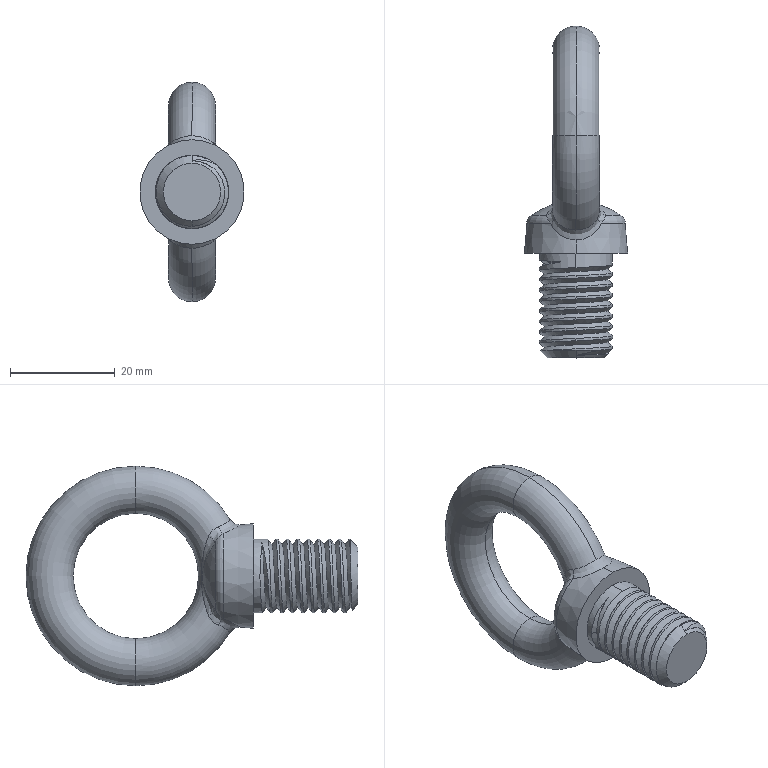Component | SolidWorks | LargeLiftingRing-2 | 1 solid | 45 faces | volume 10917 mm3 | cylinder 18 | spline 12 | torus 6 | cone 5 | plane 2 | sphere 2 | commonest cylinder face diameters 14 x18